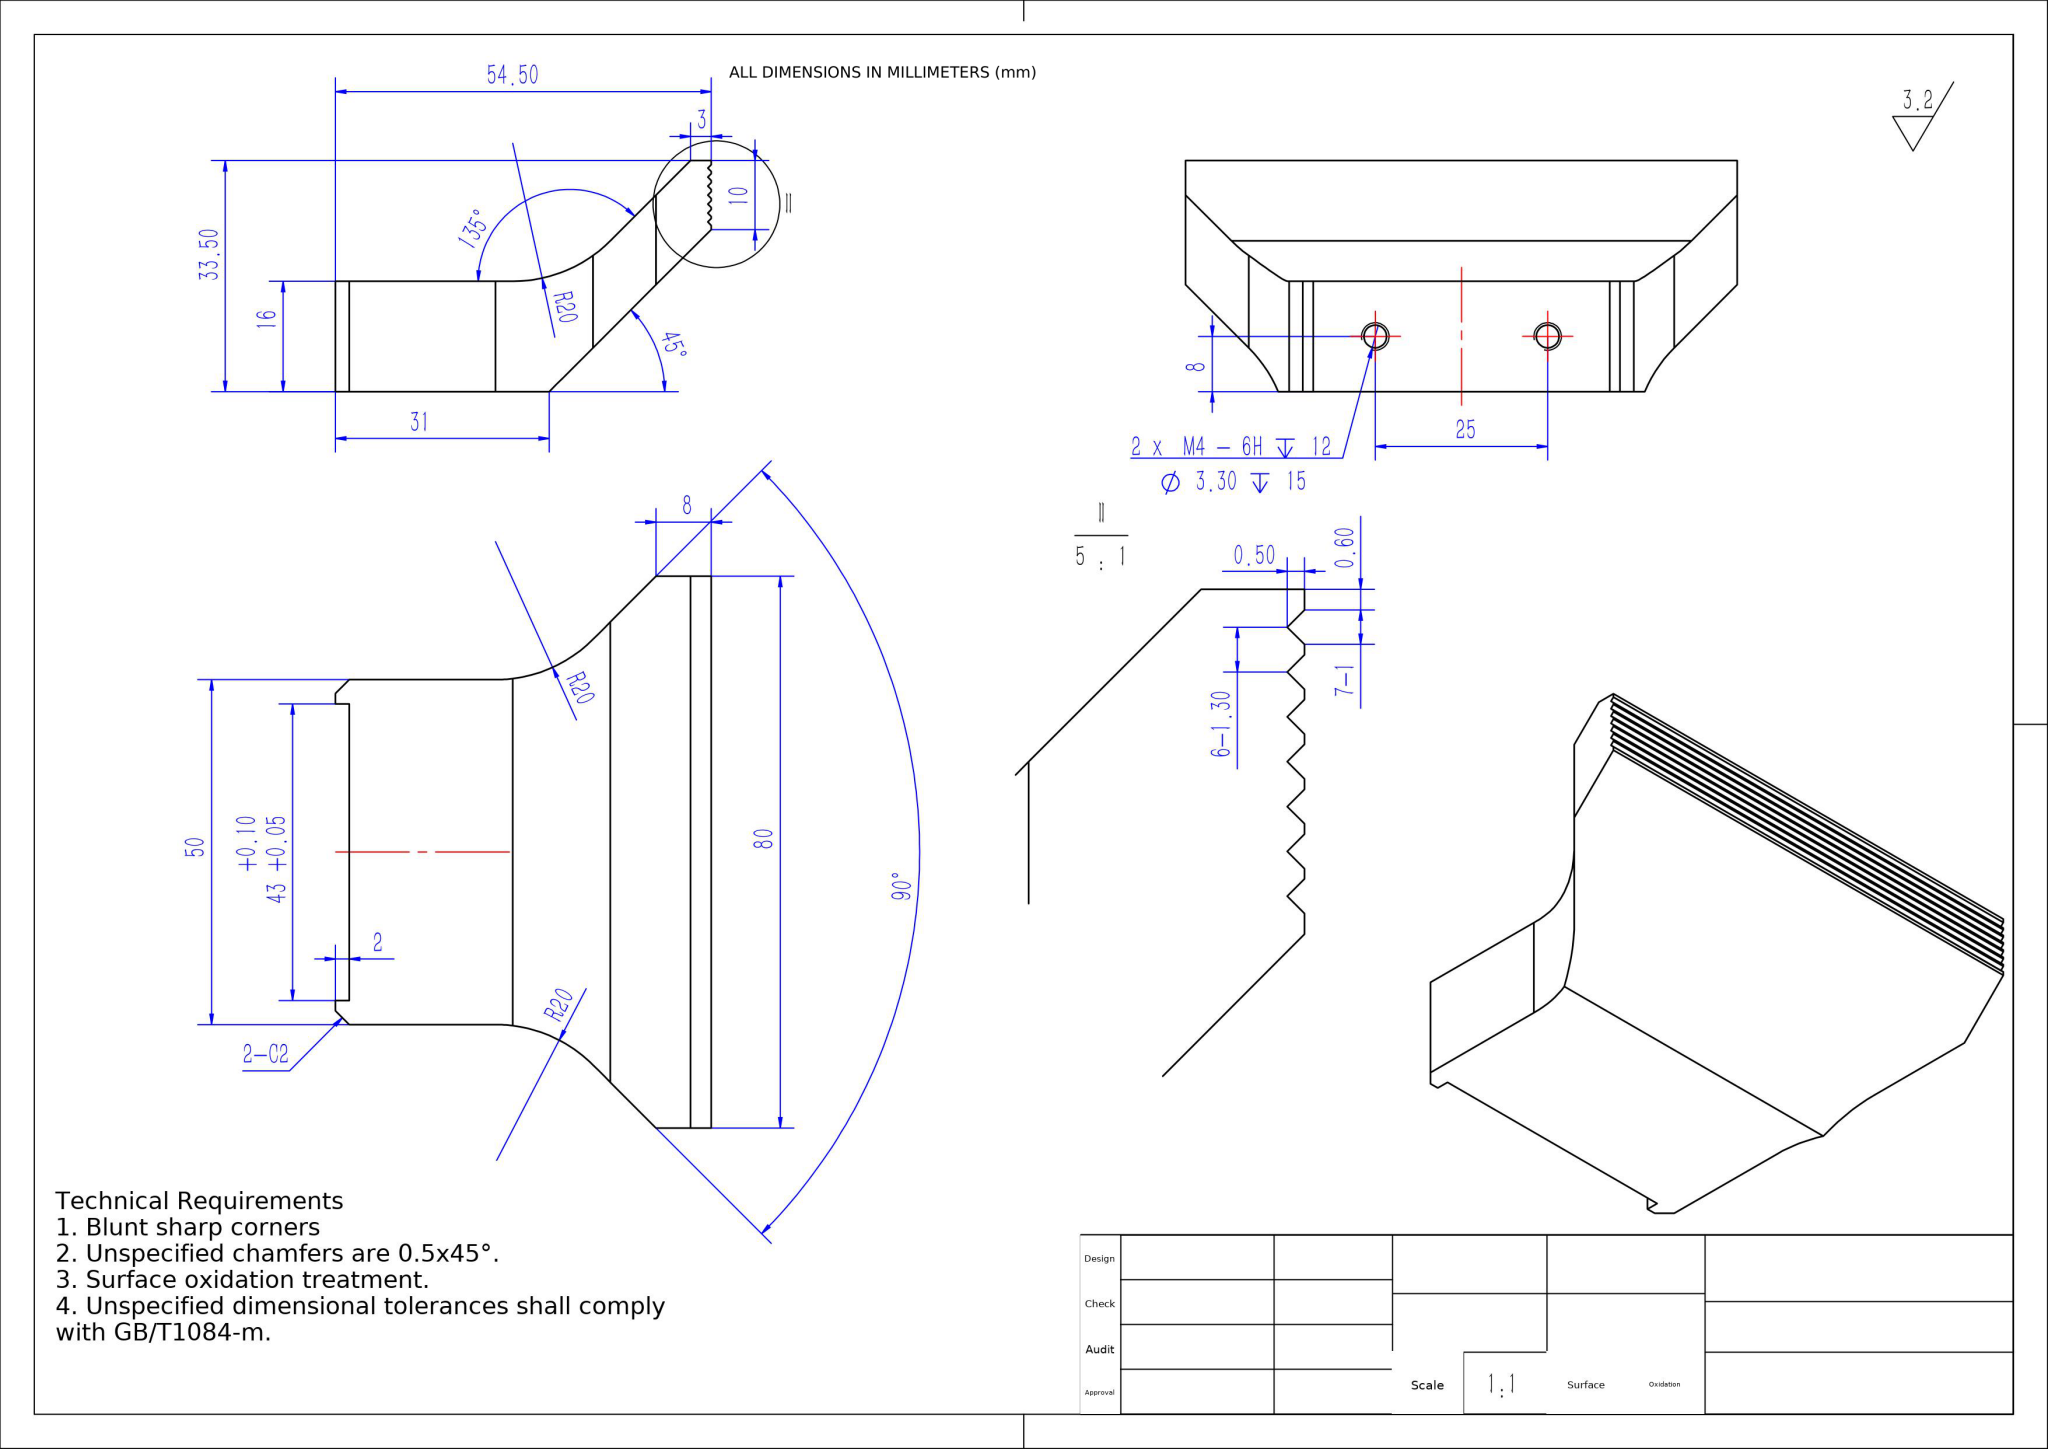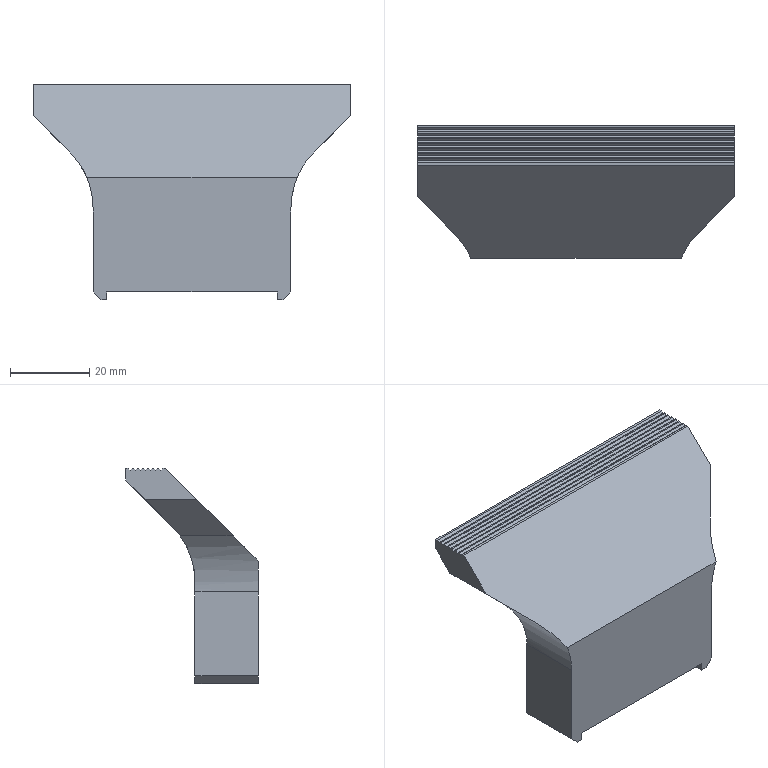Part | NX | mm | 1 solid | 51 faces | box 80 x 33.5 x 54.5 mm | volume 44926 mm3 | plane 40 | cylinder 7 | cone 4 | commonest cylinder face diameters 3.3 x4 40 x3